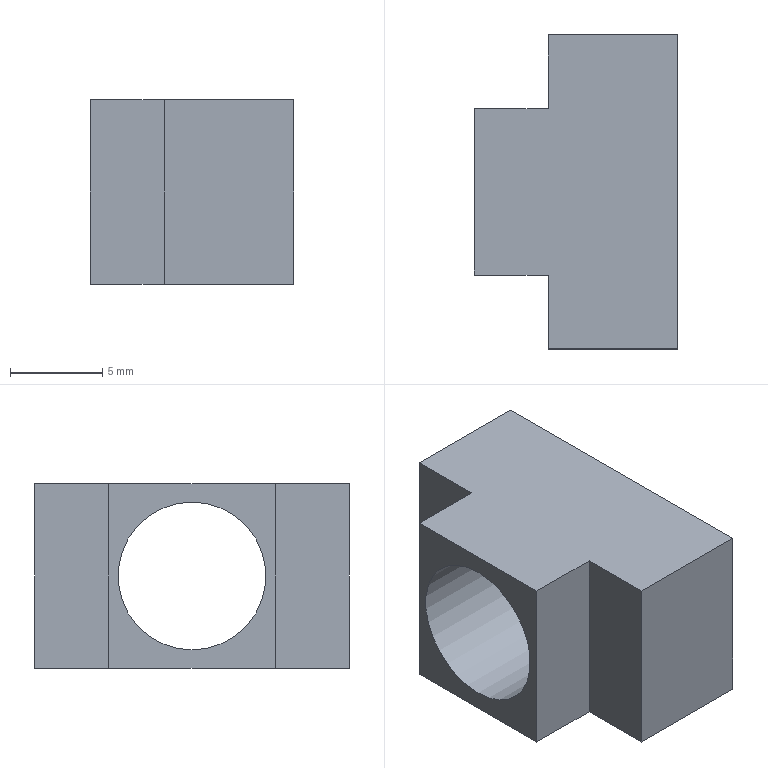Component | NX | STOP_BLOCK | 1 solid | 11 faces | box 11 x 17 x 10 mm | volume 997 mm3 | plane 10 | cylinder 1 | commonest cylinder face diameters 8 x1
STEP:
#1=CARTESIAN_POINT('',(0.,0.,0.));
#2=DIRECTION('',(0.,0.,1.));
#3=DIRECTION('',(1.,0.,0.));
#4=AXIS2_PLACEMENT_3D('',#1,#2,#3);
#5=CARTESIAN_POINT('',(-79.627,0.,11.));
#6=VERTEX_POINT('',#5);
#7=CARTESIAN_POINT('',(-79.627,0.,15.));
#8=DIRECTION('',(1.,0.,0.));
#9=DIRECTION('',(0.,0.,-1.));
#10=AXIS2_PLACEMENT_3D('',#7,#8,#9);
#11=CIRCLE('',#10,4.);
#12=CARTESIAN_POINT('',(-79.627,4.5,20.));
#13=DIRECTION('',(1.,0.,0.));
#14=DIRECTION('',(0.,0.,-1.));
#15=AXIS2_PLACEMENT_3D('',#12,#13,#14);
#16=PLANE('',#15);
#17=CARTESIAN_POINT('',(5.,-4.5));
#18=DIRECTION('',(1.,0.));
#19=AXIS2_PLACEMENT_2D('',#17,#18);
#20=CIRCLE('',#19,4.);
#21=(GEOMETRIC_REPRESENTATION_CONTEXT(2)PARAMETRIC_REPRESENTATION_CONTEXT()REPRESENTATION_CONTEXT('',''));
#22=DEFINITIONAL_REPRESENTATION('',(#20),#21);
#23=PCURVE('',#16,#22);
#24=CARTESIAN_POINT('',(-80.627,0.,15.));
#25=DIRECTION('',(1.,0.,0.));
#26=DIRECTION('',(0.,0.,-1.));
#27=AXIS2_PLACEMENT_3D('',#24,#25,#26);
#28=CYLINDRICAL_SURFACE('',#27,4.);
#29=CARTESIAN_POINT('',(0.,1.));
#30=DIRECTION('',(1.,0.));
#31=VECTOR('',#30,1.);
#32=LINE('',#29,#31);
#33=(GEOMETRIC_REPRESENTATION_CONTEXT(2)PARAMETRIC_REPRESENTATION_CONTEXT()REPRESENTATION_CONTEXT('',''));
#34=DEFINITIONAL_REPRESENTATION('',(#32),#33);
#35=PCURVE('',#28,#34);
#36=SURFACE_CURVE('',#11,(#23,#35),.PCURVE_S1.);
#37=EDGE_CURVE('',#6,#6,#36,.T.);
#38=ORIENTED_EDGE('',*,*,#37,.T.);
#39=EDGE_LOOP('',(#38));
#40=FACE_BOUND('',#39,.T.);
#41=CARTESIAN_POINT('',(-79.627,4.5,10.));
#42=VERTEX_POINT('',#41);
#43=CARTESIAN_POINT('',(-79.627,-4.5,10.));
#44=VERTEX_POINT('',#43);
#45=CARTESIAN_POINT('',(-79.627,4.5,10.));
#46=DIRECTION('',(0.,-1.,0.));
#47=VECTOR('',#46,1.);
#48=LINE('',#45,#47);
#49=CARTESIAN_POINT('',(10.,0.));
#50=DIRECTION('',(0.,-1.));
#51=VECTOR('',#50,1.);
#52=LINE('',#49,#51);
#53=(GEOMETRIC_REPRESENTATION_CONTEXT(2)PARAMETRIC_REPRESENTATION_CONTEXT()REPRESENTATION_CONTEXT('',''));
#54=DEFINITIONAL_REPRESENTATION('',(#52),#53);
#55=PCURVE('',#16,#54);
#56=CARTESIAN_POINT('',(-79.627,0.,10.));
#57=DIRECTION('',(0.,0.,1.));
#58=DIRECTION('',(1.,0.,0.));
#59=AXIS2_PLACEMENT_3D('',#56,#57,#58);
#60=PLANE('',#59);
#61=CARTESIAN_POINT('',(0.,4.5));
#62=DIRECTION('',(0.,-1.));
#63=VECTOR('',#62,1.);
#64=LINE('',#61,#63);
#65=(GEOMETRIC_REPRESENTATION_CONTEXT(2)PARAMETRIC_REPRESENTATION_CONTEXT()REPRESENTATION_CONTEXT('',''));
#66=DEFINITIONAL_REPRESENTATION('',(#64),#65);
#67=PCURVE('',#60,#66);
#68=SURFACE_CURVE('',#48,(#55,#67),.PCURVE_S1.);
#69=EDGE_CURVE('',#42,#44,#68,.T.);
#70=ORIENTED_EDGE('',*,*,#69,.T.);
#71=CARTESIAN_POINT('',(-79.627,-4.5,20.));
#72=VERTEX_POINT('',#71);
#73=CARTESIAN_POINT('',(-79.627,-4.5,20.));
#74=DIRECTION('',(0.,0.,-1.));
#75=VECTOR('',#74,1.);
#76=LINE('',#73,#75);
#77=CARTESIAN_POINT('',(0.,-9.));
#78=DIRECTION('',(1.,0.));
#79=VECTOR('',#78,1.);
#80=LINE('',#77,#79);
#81=(GEOMETRIC_REPRESENTATION_CONTEXT(2)PARAMETRIC_REPRESENTATION_CONTEXT()REPRESENTATION_CONTEXT('',''));
#82=DEFINITIONAL_REPRESENTATION('',(#80),#81);
#83=PCURVE('',#16,#82);
#84=CARTESIAN_POINT('',(-79.627,-4.5,20.));
#85=DIRECTION('',(0.,1.,0.));
#86=DIRECTION('',(0.,0.,1.));
#87=AXIS2_PLACEMENT_3D('',#84,#85,#86);
#88=PLANE('',#87);
#89=CARTESIAN_POINT('',(0.,0.));
#90=DIRECTION('',(-1.,0.));
#91=VECTOR('',#90,1.);
#92=LINE('',#89,#91);
#93=(GEOMETRIC_REPRESENTATION_CONTEXT(2)PARAMETRIC_REPRESENTATION_CONTEXT()REPRESENTATION_CONTEXT('',''));
#94=DEFINITIONAL_REPRESENTATION('',(#92),#93);
#95=PCURVE('',#88,#94);
#96=SURFACE_CURVE('',#76,(#83,#95),.PCURVE_S1.);
#97=EDGE_CURVE('',#72,#44,#96,.T.);
#98=ORIENTED_EDGE('',*,*,#97,.F.);
#99=CARTESIAN_POINT('',(-79.627,4.5,20.));
#100=VERTEX_POINT('',#99);
#101=CARTESIAN_POINT('',(-79.627,4.5,20.));
#102=DIRECTION('',(0.,-1.,0.));
#103=VECTOR('',#102,1.);
#104=LINE('',#101,#103);
#105=CARTESIAN_POINT('',(0.,0.));
#106=DIRECTION('',(0.,-1.));
#107=VECTOR('',#106,1.);
#108=LINE('',#105,#107);
#109=(GEOMETRIC_REPRESENTATION_CONTEXT(2)PARAMETRIC_REPRESENTATION_CONTEXT()REPRESENTATION_CONTEXT('',''));
#110=DEFINITIONAL_REPRESENTATION('',(#108),#109);
#111=PCURVE('',#16,#110);
#112=CARTESIAN_POINT('',(-79.627,0.,20.));
#113=DIRECTION('',(0.,0.,1.));
#114=DIRECTION('',(1.,0.,0.));
#115=AXIS2_PLACEMENT_3D('',#112,#113,#114);
#116=PLANE('',#115);
#117=CARTESIAN_POINT('',(0.,4.5));
#118=DIRECTION('',(0.,-1.));
#119=VECTOR('',#118,1.);
#120=LINE('',#117,#119);
#121=(GEOMETRIC_REPRESENTATION_CONTEXT(2)PARAMETRIC_REPRESENTATION_CONTEXT()REPRESENTATION_CONTEXT('',''));
#122=DEFINITIONAL_REPRESENTATION('',(#120),#121);
#123=PCURVE('',#116,#122);
#124=SURFACE_CURVE('',#104,(#111,#123),.PCURVE_S1.);
#125=EDGE_CURVE('',#100,#72,#124,.T.);
#126=ORIENTED_EDGE('',*,*,#125,.F.);
#127=CARTESIAN_POINT('',(-79.627,4.5,20.));
#128=DIRECTION('',(0.,0.,-1.));
#129=VECTOR('',#128,1.);
#130=LINE('',#127,#129);
#131=CARTESIAN_POINT('',(0.,0.));
#132=DIRECTION('',(1.,0.));
#133=VECTOR('',#132,1.);
#134=LINE('',#131,#133);
#135=(GEOMETRIC_REPRESENTATION_CONTEXT(2)PARAMETRIC_REPRESENTATION_CONTEXT()REPRESENTATION_CONTEXT('',''));
#136=DEFINITIONAL_REPRESENTATION('',(#134),#135);
#137=PCURVE('',#16,#136);
#138=CARTESIAN_POINT('',(-75.627,4.5,20.));
#139=DIRECTION('',(0.,-1.,0.));
#140=DIRECTION('',(0.,0.,-1.));
#141=AXIS2_PLACEMENT_3D('',#138,#139,#140);
#142=PLANE('',#141);
#143=CARTESIAN_POINT('',(0.,-4.));
#144=DIRECTION('',(1.,0.));
#145=VECTOR('',#144,1.);
#146=LINE('',#143,#145);
#147=(GEOMETRIC_REPRESENTATION_CONTEXT(2)PARAMETRIC_REPRESENTATION_CONTEXT()REPRESENTATION_CONTEXT('',''));
#148=DEFINITIONAL_REPRESENTATION('',(#146),#147);
#149=PCURVE('',#142,#148);
#150=SURFACE_CURVE('',#130,(#137,#149),.PCURVE_S1.);
#151=EDGE_CURVE('',#100,#42,#150,.T.);
#152=ORIENTED_EDGE('',*,*,#151,.T.);
#153=EDGE_LOOP('',(#70,#98,#126,#152));
#154=FACE_BOUND('',#153,.T.);
#155=ADVANCED_FACE('',(#40,#154),#16,.F.);
#156=CARTESIAN_POINT('',(-75.627,-4.5,10.));
#157=VERTEX_POINT('',#156);
#158=CARTESIAN_POINT('',(-79.627,-4.5,10.));
#159=DIRECTION('',(1.,0.,0.));
#160=VECTOR('',#159,1.);
#161=LINE('',#158,#160);
#162=CARTESIAN_POINT('',(-10.,0.));
#163=DIRECTION('',(0.,1.));
#164=VECTOR('',#163,1.);
#165=LINE('',#162,#164);
#166=(GEOMETRIC_REPRESENTATION_CONTEXT(2)PARAMETRIC_REPRESENTATION_CONTEXT()REPRESENTATION_CONTEXT('',''));
#167=DEFINITIONAL_REPRESENTATION('',(#165),#166);
#168=PCURVE('',#88,#167);
#169=CARTESIAN_POINT('',(0.,-4.5));
#170=DIRECTION('',(1.,0.));
#171=VECTOR('',#170,1.);
#172=LINE('',#169,#171);
#173=(GEOMETRIC_REPRESENTATION_CONTEXT(2)PARAMETRIC_REPRESENTATION_CONTEXT()REPRESENTATION_CONTEXT('',''));
#174=DEFINITIONAL_REPRESENTATION('',(#172),#173);
#175=PCURVE('',#60,#174);
#176=SURFACE_CURVE('',#161,(#168,#175),.PCURVE_S1.);
#177=EDGE_CURVE('',#44,#157,#176,.T.);
#178=ORIENTED_EDGE('',*,*,#177,.T.);
#179=CARTESIAN_POINT('',(-75.627,-4.5,20.));
#180=VERTEX_POINT('',#179);
#181=CARTESIAN_POINT('',(-75.627,-4.5,20.));
#182=DIRECTION('',(0.,0.,-1.));
#183=VECTOR('',#182,1.);
#184=LINE('',#181,#183);
#185=CARTESIAN_POINT('',(0.,4.));
#186=DIRECTION('',(-1.,0.));
#187=VECTOR('',#186,1.);
#188=LINE('',#185,#187);
#189=(GEOMETRIC_REPRESENTATION_CONTEXT(2)PARAMETRIC_REPRESENTATION_CONTEXT()REPRESENTATION_CONTEXT('',''));
#190=DEFINITIONAL_REPRESENTATION('',(#188),#189);
#191=PCURVE('',#88,#190);
#192=CARTESIAN_POINT('',(-75.627,-4.5,20.));
#193=DIRECTION('',(1.,0.,0.));
#194=DIRECTION('',(0.,0.,-1.));
#195=AXIS2_PLACEMENT_3D('',#192,#193,#194);
#196=PLANE('',#195);
#197=CARTESIAN_POINT('',(0.,0.));
#198=DIRECTION('',(1.,0.));
#199=VECTOR('',#198,1.);
#200=LINE('',#197,#199);
#201=(GEOMETRIC_REPRESENTATION_CONTEXT(2)PARAMETRIC_REPRESENTATION_CONTEXT()REPRESENTATION_CONTEXT('',''));
#202=DEFINITIONAL_REPRESENTATION('',(#200),#201);
#203=PCURVE('',#196,#202);
#204=SURFACE_CURVE('',#184,(#191,#203),.PCURVE_S1.);
#205=EDGE_CURVE('',#180,#157,#204,.T.);
#206=ORIENTED_EDGE('',*,*,#205,.F.);
#207=CARTESIAN_POINT('',(-79.627,-4.5,20.));
#208=DIRECTION('',(1.,0.,0.));
#209=VECTOR('',#208,1.);
#210=LINE('',#207,#209);
#211=CARTESIAN_POINT('',(0.,0.));
#212=DIRECTION('',(0.,1.));
#213=VECTOR('',#212,1.);
#214=LINE('',#211,#213);
#215=(GEOMETRIC_REPRESENTATION_CONTEXT(2)PARAMETRIC_REPRESENTATION_CONTEXT()REPRESENTATION_CONTEXT('',''));
#216=DEFINITIONAL_REPRESENTATION('',(#214),#215);
#217=PCURVE('',#88,#216);
#218=CARTESIAN_POINT('',(0.,-4.5));
#219=DIRECTION('',(1.,0.));
#220=VECTOR('',#219,1.);
#221=LINE('',#218,#220);
#222=(GEOMETRIC_REPRESENTATION_CONTEXT(2)PARAMETRIC_REPRESENTATION_CONTEXT()REPRESENTATION_CONTEXT('',''));
#223=DEFINITIONAL_REPRESENTATION('',(#221),#222);
#224=PCURVE('',#116,#223);
#225=SURFACE_CURVE('',#210,(#217,#224),.PCURVE_S1.);
#226=EDGE_CURVE('',#72,#180,#225,.T.);
#227=ORIENTED_EDGE('',*,*,#226,.F.);
#228=ORIENTED_EDGE('',*,*,#97,.T.);
#229=EDGE_LOOP('',(#178,#206,#227,#228));
#230=FACE_BOUND('',#229,.T.);
#231=ADVANCED_FACE('',(#230),#88,.F.);
#232=CARTESIAN_POINT('',(-75.627,-8.5,10.));
#233=VERTEX_POINT('',#232);
#234=CARTESIAN_POINT('',(-75.627,-4.5,10.));
#235=DIRECTION('',(0.,-1.,0.));
#236=VECTOR('',#235,1.);
#237=LINE('',#234,#236);
#238=CARTESIAN_POINT('',(10.,0.));
#239=DIRECTION('',(0.,-1.));
#240=VECTOR('',#239,1.);
#241=LINE('',#238,#240);
#242=(GEOMETRIC_REPRESENTATION_CONTEXT(2)PARAMETRIC_REPRESENTATION_CONTEXT()REPRESENTATION_CONTEXT('',''));
#243=DEFINITIONAL_REPRESENTATION('',(#241),#242);
#244=PCURVE('',#196,#243);
#245=CARTESIAN_POINT('',(4.,-4.5));
#246=DIRECTION('',(0.,-1.));
#247=VECTOR('',#246,1.);
#248=LINE('',#245,#247);
#249=(GEOMETRIC_REPRESENTATION_CONTEXT(2)PARAMETRIC_REPRESENTATION_CONTEXT()REPRESENTATION_CONTEXT('',''));
#250=DEFINITIONAL_REPRESENTATION('',(#248),#249);
#251=PCURVE('',#60,#250);
#252=SURFACE_CURVE('',#237,(#244,#251),.PCURVE_S1.);
#253=EDGE_CURVE('',#157,#233,#252,.T.);
#254=ORIENTED_EDGE('',*,*,#253,.T.);
#255=CARTESIAN_POINT('',(-75.627,-8.5,20.));
#256=VERTEX_POINT('',#255);
#257=CARTESIAN_POINT('',(-75.627,-8.5,20.));
#258=DIRECTION('',(0.,0.,-1.));
#259=VECTOR('',#258,1.);
#260=LINE('',#257,#259);
#261=CARTESIAN_POINT('',(0.,-4.));
#262=DIRECTION('',(1.,0.));
#263=VECTOR('',#262,1.);
#264=LINE('',#261,#263);
#265=(GEOMETRIC_REPRESENTATION_CONTEXT(2)PARAMETRIC_REPRESENTATION_CONTEXT()REPRESENTATION_CONTEXT('',''));
#266=DEFINITIONAL_REPRESENTATION('',(#264),#265);
#267=PCURVE('',#196,#266);
#268=CARTESIAN_POINT('',(-75.627,-8.5,20.));
#269=DIRECTION('',(0.,1.,0.));
#270=DIRECTION('',(0.,0.,1.));
#271=AXIS2_PLACEMENT_3D('',#268,#269,#270);
#272=PLANE('',#271);
#273=CARTESIAN_POINT('',(0.,0.));
#274=DIRECTION('',(-1.,0.));
#275=VECTOR('',#274,1.);
#276=LINE('',#273,#275);
#277=(GEOMETRIC_REPRESENTATION_CONTEXT(2)PARAMETRIC_REPRESENTATION_CONTEXT()REPRESENTATION_CONTEXT('',''));
#278=DEFINITIONAL_REPRESENTATION('',(#276),#277);
#279=PCURVE('',#272,#278);
#280=SURFACE_CURVE('',#260,(#267,#279),.PCURVE_S1.);
#281=EDGE_CURVE('',#256,#233,#280,.T.);
#282=ORIENTED_EDGE('',*,*,#281,.F.);
#283=CARTESIAN_POINT('',(-75.627,-4.5,20.));
#284=DIRECTION('',(0.,-1.,0.));
#285=VECTOR('',#284,1.);
#286=LINE('',#283,#285);
#287=CARTESIAN_POINT('',(0.,0.));
#288=DIRECTION('',(0.,-1.));
#289=VECTOR('',#288,1.);
#290=LINE('',#287,#289);
#291=(GEOMETRIC_REPRESENTATION_CONTEXT(2)PARAMETRIC_REPRESENTATION_CONTEXT()REPRESENTATION_CONTEXT('',''));
#292=DEFINITIONAL_REPRESENTATION('',(#290),#291);
#293=PCURVE('',#196,#292);
#294=CARTESIAN_POINT('',(4.,-4.5));
#295=DIRECTION('',(0.,-1.));
#296=VECTOR('',#295,1.);
#297=LINE('',#294,#296);
#298=(GEOMETRIC_REPRESENTATION_CONTEXT(2)PARAMETRIC_REPRESENTATION_CONTEXT()REPRESENTATION_CONTEXT('',''));
#299=DEFINITIONAL_REPRESENTATION('',(#297),#298);
#300=PCURVE('',#116,#299);
#301=SURFACE_CURVE('',#286,(#293,#300),.PCURVE_S1.);
#302=EDGE_CURVE('',#180,#256,#301,.T.);
#303=ORIENTED_EDGE('',*,*,#302,.F.);
#304=ORIENTED_EDGE('',*,*,#205,.T.);
#305=EDGE_LOOP('',(#254,#282,#303,#304));
#306=FACE_BOUND('',#305,.T.);
#307=ADVANCED_FACE('',(#306),#196,.F.);
#308=CARTESIAN_POINT('',(-68.627,-8.5,10.));
#309=VERTEX_POINT('',#308);
#310=CARTESIAN_POINT('',(-75.627,-8.5,10.));
#311=DIRECTION('',(1.,0.,0.));
#312=VECTOR('',#311,1.);
#313=LINE('',#310,#312);
#314=CARTESIAN_POINT('',(-10.,0.));
#315=DIRECTION('',(0.,1.));
#316=VECTOR('',#315,1.);
#317=LINE('',#314,#316);
#318=(GEOMETRIC_REPRESENTATION_CONTEXT(2)PARAMETRIC_REPRESENTATION_CONTEXT()REPRESENTATION_CONTEXT('',''));
#319=DEFINITIONAL_REPRESENTATION('',(#317),#318);
#320=PCURVE('',#272,#319);
#321=CARTESIAN_POINT('',(4.,-8.5));
#322=DIRECTION('',(1.,0.));
#323=VECTOR('',#322,1.);
#324=LINE('',#321,#323);
#325=(GEOMETRIC_REPRESENTATION_CONTEXT(2)PARAMETRIC_REPRESENTATION_CONTEXT()REPRESENTATION_CONTEXT('',''));
#326=DEFINITIONAL_REPRESENTATION('',(#324),#325);
#327=PCURVE('',#60,#326);
#328=SURFACE_CURVE('',#313,(#320,#327),.PCURVE_S1.);
#329=EDGE_CURVE('',#233,#309,#328,.T.);
#330=ORIENTED_EDGE('',*,*,#329,.T.);
#331=CARTESIAN_POINT('',(-68.627,-8.5,20.));
#332=VERTEX_POINT('',#331);
#333=CARTESIAN_POINT('',(-68.627,-8.5,20.));
#334=DIRECTION('',(0.,0.,-1.));
#335=VECTOR('',#334,1.);
#336=LINE('',#333,#335);
#337=CARTESIAN_POINT('',(0.,7.));
#338=DIRECTION('',(-1.,0.));
#339=VECTOR('',#338,1.);
#340=LINE('',#337,#339);
#341=(GEOMETRIC_REPRESENTATION_CONTEXT(2)PARAMETRIC_REPRESENTATION_CONTEXT()REPRESENTATION_CONTEXT('',''));
#342=DEFINITIONAL_REPRESENTATION('',(#340),#341);
#343=PCURVE('',#272,#342);
#344=CARTESIAN_POINT('',(-68.627,-8.5,20.));
#345=DIRECTION('',(-1.,0.,0.));
#346=DIRECTION('',(0.,0.,1.));
#347=AXIS2_PLACEMENT_3D('',#344,#345,#346);
#348=PLANE('',#347);
#349=CARTESIAN_POINT('',(0.,0.));
#350=DIRECTION('',(-1.,0.));
#351=VECTOR('',#350,1.);
#352=LINE('',#349,#351);
#353=(GEOMETRIC_REPRESENTATION_CONTEXT(2)PARAMETRIC_REPRESENTATION_CONTEXT()REPRESENTATION_CONTEXT('',''));
#354=DEFINITIONAL_REPRESENTATION('',(#352),#353);
#355=PCURVE('',#348,#354);
#356=SURFACE_CURVE('',#336,(#343,#355),.PCURVE_S1.);
#357=EDGE_CURVE('',#332,#309,#356,.T.);
#358=ORIENTED_EDGE('',*,*,#357,.F.);
#359=CARTESIAN_POINT('',(-75.627,-8.5,20.));
#360=DIRECTION('',(1.,0.,0.));
#361=VECTOR('',#360,1.);
#362=LINE('',#359,#361);
#363=CARTESIAN_POINT('',(0.,0.));
#364=DIRECTION('',(0.,1.));
#365=VECTOR('',#364,1.);
#366=LINE('',#363,#365);
#367=(GEOMETRIC_REPRESENTATION_CONTEXT(2)PARAMETRIC_REPRESENTATION_CONTEXT()REPRESENTATION_CONTEXT('',''));
#368=DEFINITIONAL_REPRESENTATION('',(#366),#367);
#369=PCURVE('',#272,#368);
#370=CARTESIAN_POINT('',(4.,-8.5));
#371=DIRECTION('',(1.,0.));
#372=VECTOR('',#371,1.);
#373=LINE('',#370,#372);
#374=(GEOMETRIC_REPRESENTATION_CONTEXT(2)PARAMETRIC_REPRESENTATION_CONTEXT()REPRESENTATION_CONTEXT('',''));
#375=DEFINITIONAL_REPRESENTATION('',(#373),#374);
#376=PCURVE('',#116,#375);
#377=SURFACE_CURVE('',#362,(#369,#376),.PCURVE_S1.);
#378=EDGE_CURVE('',#256,#332,#377,.T.);
#379=ORIENTED_EDGE('',*,*,#378,.F.);
#380=ORIENTED_EDGE('',*,*,#281,.T.);
#381=EDGE_LOOP('',(#330,#358,#379,#380));
#382=FACE_BOUND('',#381,.T.);
#383=ADVANCED_FACE('',(#382),#272,.F.);
#384=CARTESIAN_POINT('',(-68.627,0.,19.));
#385=VERTEX_POINT('',#384);
#386=CARTESIAN_POINT('',(-68.627,0.,11.));
#387=VERTEX_POINT('',#386);
#388=CARTESIAN_POINT('',(-68.627,0.,15.));
#389=DIRECTION('',(-1.,0.,0.));
#390=DIRECTION('',(0.,0.,1.));
#391=AXIS2_PLACEMENT_3D('',#388,#389,#390);
#392=CIRCLE('',#391,4.);
#393=CARTESIAN_POINT('',(-5.,8.5));
#394=DIRECTION('',(1.,0.));
#395=AXIS2_PLACEMENT_2D('',#393,#394);
#396=CIRCLE('',#395,4.);
#397=(GEOMETRIC_REPRESENTATION_CONTEXT(2)PARAMETRIC_REPRESENTATION_CONTEXT()REPRESENTATION_CONTEXT('',''));
#398=DEFINITIONAL_REPRESENTATION('',(#396),#397);
#399=PCURVE('',#348,#398);
#400=CARTESIAN_POINT('',(3.142,12.));
#401=DIRECTION('',(-1.,0.));
#402=VECTOR('',#401,1.);
#403=LINE('',#400,#402);
#404=(GEOMETRIC_REPRESENTATION_CONTEXT(2)PARAMETRIC_REPRESENTATION_CONTEXT()REPRESENTATION_CONTEXT('',''));
#405=DEFINITIONAL_REPRESENTATION('',(#403),#404);
#406=PCURVE('',#28,#405);
#407=SURFACE_CURVE('',#392,(#399,#406),.PCURVE_S1.);
#408=EDGE_CURVE('',#385,#387,#407,.T.);
#409=ORIENTED_EDGE('',*,*,#408,.T.);
#410=CARTESIAN_POINT('',(-68.627,0.,15.));
#411=DIRECTION('',(-1.,0.,0.));
#412=DIRECTION('',(0.,0.,1.));
#413=AXIS2_PLACEMENT_3D('',#410,#411,#412);
#414=CIRCLE('',#413,4.);
#415=CARTESIAN_POINT('',(-5.,8.5));
#416=DIRECTION('',(1.,0.));
#417=AXIS2_PLACEMENT_2D('',#415,#416);
#418=CIRCLE('',#417,4.);
#419=(GEOMETRIC_REPRESENTATION_CONTEXT(2)PARAMETRIC_REPRESENTATION_CONTEXT()REPRESENTATION_CONTEXT('',''));
#420=DEFINITIONAL_REPRESENTATION('',(#418),#419);
#421=PCURVE('',#348,#420);
#422=CARTESIAN_POINT('',(9.425,12.));
#423=DIRECTION('',(-1.,0.));
#424=VECTOR('',#423,1.);
#425=LINE('',#422,#424);
#426=(GEOMETRIC_REPRESENTATION_CONTEXT(2)PARAMETRIC_REPRESENTATION_CONTEXT()REPRESENTATION_CONTEXT('',''));
#427=DEFINITIONAL_REPRESENTATION('',(#425),#426);
#428=PCURVE('',#28,#427);
#429=SURFACE_CURVE('',#414,(#421,#428),.PCURVE_S1.);
#430=EDGE_CURVE('',#387,#385,#429,.T.);
#431=ORIENTED_EDGE('',*,*,#430,.T.);
#432=EDGE_LOOP('',(#409,#431));
#433=FACE_BOUND('',#432,.T.);
#434=CARTESIAN_POINT('',(-68.627,8.5,10.));
#435=VERTEX_POINT('',#434);
#436=CARTESIAN_POINT('',(-68.627,-8.5,10.));
#437=DIRECTION('',(0.,1.,0.));
#438=VECTOR('',#437,1.);
#439=LINE('',#436,#438);
#440=CARTESIAN_POINT('',(-10.,0.));
#441=DIRECTION('',(0.,1.));
#442=VECTOR('',#441,1.);
#443=LINE('',#440,#442);
#444=(GEOMETRIC_REPRESENTATION_CONTEXT(2)PARAMETRIC_REPRESENTATION_CONTEXT()REPRESENTATION_CONTEXT('',''));
#445=DEFINITIONAL_REPRESENTATION('',(#443),#444);
#446=PCURVE('',#348,#445);
#447=CARTESIAN_POINT('',(11.,-8.5));
#448=DIRECTION('',(0.,1.));
#449=VECTOR('',#448,1.);
#450=LINE('',#447,#449);
#451=(GEOMETRIC_REPRESENTATION_CONTEXT(2)PARAMETRIC_REPRESENTATION_CONTEXT()REPRESENTATION_CONTEXT('',''));
#452=DEFINITIONAL_REPRESENTATION('',(#450),#451);
#453=PCURVE('',#60,#452);
#454=SURFACE_CURVE('',#439,(#446,#453),.PCURVE_S1.);
#455=EDGE_CURVE('',#309,#435,#454,.T.);
#456=ORIENTED_EDGE('',*,*,#455,.T.);
#457=CARTESIAN_POINT('',(-68.627,8.5,20.));
#458=VERTEX_POINT('',#457);
#459=CARTESIAN_POINT('',(-68.627,8.5,20.));
#460=DIRECTION('',(0.,0.,-1.));
#461=VECTOR('',#460,1.);
#462=LINE('',#459,#461);
#463=CARTESIAN_POINT('',(0.,17.));
#464=DIRECTION('',(-1.,0.));
#465=VECTOR('',#464,1.);
#466=LINE('',#463,#465);
#467=(GEOMETRIC_REPRESENTATION_CONTEXT(2)PARAMETRIC_REPRESENTATION_CONTEXT()REPRESENTATION_CONTEXT('',''));
#468=DEFINITIONAL_REPRESENTATION('',(#466),#467);
#469=PCURVE('',#348,#468);
#470=CARTESIAN_POINT('',(-68.627,8.5,20.));
#471=DIRECTION('',(0.,-1.,0.));
#472=DIRECTION('',(0.,0.,-1.));
#473=AXIS2_PLACEMENT_3D('',#470,#471,#472);
#474=PLANE('',#473);
#475=CARTESIAN_POINT('',(0.,0.));
#476=DIRECTION('',(1.,0.));
#477=VECTOR('',#476,1.);
#478=LINE('',#475,#477);
#479=(GEOMETRIC_REPRESENTATION_CONTEXT(2)PARAMETRIC_REPRESENTATION_CONTEXT()REPRESENTATION_CONTEXT('',''));
#480=DEFINITIONAL_REPRESENTATION('',(#478),#479);
#481=PCURVE('',#474,#480);
#482=SURFACE_CURVE('',#462,(#469,#481),.PCURVE_S1.);
#483=EDGE_CURVE('',#458,#435,#482,.T.);
#484=ORIENTED_EDGE('',*,*,#483,.F.);
#485=CARTESIAN_POINT('',(-68.627,-8.5,20.));
#486=DIRECTION('',(0.,1.,0.));
#487=VECTOR('',#486,1.);
#488=LINE('',#485,#487);
#489=CARTESIAN_POINT('',(0.,0.));
#490=DIRECTION('',(0.,1.));
#491=VECTOR('',#490,1.);
#492=LINE('',#489,#491);
#493=(GEOMETRIC_REPRESENTATION_CONTEXT(2)PARAMETRIC_REPRESENTATION_CONTEXT()REPRESENTATION_CONTEXT('',''));
#494=DEFINITIONAL_REPRESENTATION('',(#492),#493);
#495=PCURVE('',#348,#494);
#496=CARTESIAN_POINT('',(11.,-8.5));
#497=DIRECTION('',(0.,1.));
#498=VECTOR('',#497,1.);
#499=LINE('',#496,#498);
#500=(GEOMETRIC_REPRESENTATION_CONTEXT(2)PARAMETRIC_REPRESENTATION_CONTEXT()REPRESENTATION_CONTEXT('',''));
#501=DEFINITIONAL_REPRESENTATION('',(#499),#500);
#502=PCURVE('',#116,#501);
#503=SURFACE_CURVE('',#488,(#495,#502),.PCURVE_S1.);
#504=EDGE_CURVE('',#332,#458,#503,.T.);
#505=ORIENTED_EDGE('',*,*,#504,.F.);
#506=ORIENTED_EDGE('',*,*,#357,.T.);
#507=EDGE_LOOP('',(#456,#484,#505,#506));
#508=FACE_BOUND('',#507,.T.);
#509=ADVANCED_FACE('',(#433,#508),#348,.F.);
#510=CARTESIAN_POINT('',(-75.627,8.5,10.));
#511=VERTEX_POINT('',#510);
#512=CARTESIAN_POINT('',(-68.627,8.5,10.));
#513=DIRECTION('',(-1.,0.,0.));
#514=VECTOR('',#513,1.);
#515=LINE('',#512,#514);
#516=CARTESIAN_POINT('',(10.,0.));
#517=DIRECTION('',(0.,-1.));
#518=VECTOR('',#517,1.);
#519=LINE('',#516,#518);
#520=(GEOMETRIC_REPRESENTATION_CONTEXT(2)PARAMETRIC_REPRESENTATION_CONTEXT()REPRESENTATION_CONTEXT('',''));
#521=DEFINITIONAL_REPRESENTATION('',(#519),#520);
#522=PCURVE('',#474,#521);
#523=CARTESIAN_POINT('',(11.,8.5));
#524=DIRECTION('',(-1.,0.));
#525=VECTOR('',#524,1.);
#526=LINE('',#523,#525);
#527=(GEOMETRIC_REPRESENTATION_CONTEXT(2)PARAMETRIC_REPRESENTATION_CONTEXT()REPRESENTATION_CONTEXT('',''));
#528=DEFINITIONAL_REPRESENTATION('',(#526),#527);
#529=PCURVE('',#60,#528);
#530=SURFACE_CURVE('',#515,(#522,#529),.PCURVE_S1.);
#531=EDGE_CURVE('',#435,#511,#530,.T.);
#532=ORIENTED_EDGE('',*,*,#531,.T.);
#533=CARTESIAN_POINT('',(-75.627,8.5,20.));
#534=VERTEX_POINT('',#533);
#535=CARTESIAN_POINT('',(-75.627,8.5,20.));
#536=DIRECTION('',(0.,0.,-1.));
#537=VECTOR('',#536,1.);
#538=LINE('',#535,#537);
#539=CARTESIAN_POINT('',(0.,-7.));
#540=DIRECTION('',(1.,0.));
#541=VECTOR('',#540,1.);
#542=LINE('',#539,#541);
#543=(GEOMETRIC_REPRESENTATION_CONTEXT(2)PARAMETRIC_REPRESENTATION_CONTEXT()REPRESENTATION_CONTEXT('',''));
#544=DEFINITIONAL_REPRESENTATION('',(#542),#543);
#545=PCURVE('',#474,#544);
#546=CARTESIAN_POINT('',(-75.627,8.5,20.));
#547=DIRECTION('',(1.,0.,0.));
#548=DIRECTION('',(0.,0.,-1.));
#549=AXIS2_PLACEMENT_3D('',#546,#547,#548);
#550=PLANE('',#549);
#551=CARTESIAN_POINT('',(0.,0.));
#552=DIRECTION('',(1.,0.));
#553=VECTOR('',#552,1.);
#554=LINE('',#551,#553);
#555=(GEOMETRIC_REPRESENTATION_CONTEXT(2)PARAMETRIC_REPRESENTATION_CONTEXT()REPRESENTATION_CONTEXT('',''));
#556=DEFINITIONAL_REPRESENTATION('',(#554),#555);
#557=PCURVE('',#550,#556);
#558=SURFACE_CURVE('',#538,(#545,#557),.PCURVE_S1.);
#559=EDGE_CURVE('',#534,#511,#558,.T.);
#560=ORIENTED_EDGE('',*,*,#559,.F.);
#561=CARTESIAN_POINT('',(-68.627,8.5,20.));
#562=DIRECTION('',(-1.,0.,0.));
#563=VECTOR('',#562,1.);
#564=LINE('',#561,#563);
#565=CARTESIAN_POINT('',(0.,0.));
#566=DIRECTION('',(0.,-1.));
#567=VECTOR('',#566,1.);
#568=LINE('',#565,#567);
#569=(GEOMETRIC_REPRESENTATION_CONTEXT(2)PARAMETRIC_REPRESENTATION_CONTEXT()REPRESENTATION_CONTEXT('',''));
#570=DEFINITIONAL_REPRESENTATION('',(#568),#569);
#571=PCURVE('',#474,#570);
#572=CARTESIAN_POINT('',(11.,8.5));
#573=DIRECTION('',(-1.,0.));
#574=VECTOR('',#573,1.);
#575=LINE('',#572,#574);
#576=(GEOMETRIC_REPRESENTATION_CONTEXT(2)PARAMETRIC_REPRESENTATION_CONTEXT()REPRESENTATION_CONTEXT('',''));
#577=DEFINITIONAL_REPRESENTATION('',(#575),#576);
#578=PCURVE('',#116,#577);
#579=SURFACE_CURVE('',#564,(#571,#578),.PCURVE_S1.);
#580=EDGE_CURVE('',#458,#534,#579,.T.);
#581=ORIENTED_EDGE('',*,*,#580,.F.);
#582=ORIENTED_EDGE('',*,*,#483,.T.);
#583=EDGE_LOOP('',(#532,#560,#581,#582));
#584=FACE_BOUND('',#583,.T.);
#585=ADVANCED_FACE('',(#584),#474,.F.);
#586=CARTESIAN_POINT('',(-75.627,4.5,10.));
#587=VERTEX_POINT('',#586);
#588=CARTESIAN_POINT('',(-75.627,8.5,10.));
#589=DIRECTION('',(0.,-1.,0.));
#590=VECTOR('',#589,1.);
#591=LINE('',#588,#590);
#592=CARTESIAN_POINT('',(10.,0.));
#593=DIRECTION('',(0.,-1.));
#594=VECTOR('',#593,1.);
#595=LINE('',#592,#594);
#596=(GEOMETRIC_REPRESENTATION_CONTEXT(2)PARAMETRIC_REPRESENTATION_CONTEXT()REPRESENTATION_CONTEXT('',''));
#597=DEFINITIONAL_REPRESENTATION('',(#595),#596);
#598=PCURVE('',#550,#597);
#599=CARTESIAN_POINT('',(4.,8.5));
#600=DIRECTION('',(0.,-1.));
#601=VECTOR('',#600,1.);
#602=LINE('',#599,#601);
#603=(GEOMETRIC_REPRESENTATION_CONTEXT(2)PARAMETRIC_REPRESENTATION_CONTEXT()REPRESENTATION_CONTEXT('',''));
#604=DEFINITIONAL_REPRESENTATION('',(#602),#603);
#605=PCURVE('',#60,#604);
#606=SURFACE_CURVE('',#591,(#598,#605),.PCURVE_S1.);
#607=EDGE_CURVE('',#511,#587,#606,.T.);
#608=ORIENTED_EDGE('',*,*,#607,.T.);
#609=CARTESIAN_POINT('',(-75.627,4.5,20.));
#610=VERTEX_POINT('',#609);
#611=CARTESIAN_POINT('',(-75.627,4.5,20.));
#612=DIRECTION('',(0.,0.,-1.));
#613=VECTOR('',#612,1.);
#614=LINE('',#611,#613);
#615=CARTESIAN_POINT('',(0.,-4.));
#616=DIRECTION('',(1.,0.));
#617=VECTOR('',#616,1.);
#618=LINE('',#615,#617);
#619=(GEOMETRIC_REPRESENTATION_CONTEXT(2)PARAMETRIC_REPRESENTATION_CONTEXT()REPRESENTATION_CONTEXT('',''));
#620=DEFINITIONAL_REPRESENTATION('',(#618),#619);
#621=PCURVE('',#550,#620);
#622=CARTESIAN_POINT('',(0.,0.));
#623=DIRECTION('',(1.,0.));
#624=VECTOR('',#623,1.);
#625=LINE('',#622,#624);
#626=(GEOMETRIC_REPRESENTATION_CONTEXT(2)PARAMETRIC_REPRESENTATION_CONTEXT()REPRESENTATION_CONTEXT('',''));
#627=DEFINITIONAL_REPRESENTATION('',(#625),#626);
#628=PCURVE('',#142,#627);
#629=SURFACE_CURVE('',#614,(#621,#628),.PCURVE_S1.);
#630=EDGE_CURVE('',#610,#587,#629,.T.);
#631=ORIENTED_EDGE('',*,*,#630,.F.);
#632=CARTESIAN_POINT('',(-75.627,8.5,20.));
#633=DIRECTION('',(0.,-1.,0.));
#634=VECTOR('',#633,1.);
#635=LINE('',#632,#634);
#636=CARTESIAN_POINT('',(0.,0.));
#637=DIRECTION('',(0.,-1.));
#638=VECTOR('',#637,1.);
#639=LINE('',#636,#638);
#640=(GEOMETRIC_REPRESENTATION_CONTEXT(2)PARAMETRIC_REPRESENTATION_CONTEXT()REPRESENTATION_CONTEXT('',''));
#641=DEFINITIONAL_REPRESENTATION('',(#639),#640);
#642=PCURVE('',#550,#641);
#643=CARTESIAN_POINT('',(4.,8.5));
#644=DIRECTION('',(0.,-1.));
#645=VECTOR('',#644,1.);
#646=LINE('',#643,#645);
#647=(GEOMETRIC_REPRESENTATION_CONTEXT(2)PARAMETRIC_REPRESENTATION_CONTEXT()REPRESENTATION_CONTEXT('',''));
#648=DEFINITIONAL_REPRESENTATION('',(#646),#647);
#649=PCURVE('',#116,#648);
#650=SURFACE_CURVE('',#635,(#642,#649),.PCURVE_S1.);
#651=EDGE_CURVE('',#534,#610,#650,.T.);
#652=ORIENTED_EDGE('',*,*,#651,.F.);
#653=ORIENTED_EDGE('',*,*,#559,.T.);
#654=EDGE_LOOP('',(#608,#631,#652,#653));
#655=FACE_BOUND('',#654,.T.);
#656=ADVANCED_FACE('',(#655),#550,.F.);
#657=CARTESIAN_POINT('',(-75.627,4.5,10.));
#658=DIRECTION('',(-1.,0.,0.));
#659=VECTOR('',#658,1.);
#660=LINE('',#657,#659);
#661=CARTESIAN_POINT('',(10.,0.));
#662=DIRECTION('',(0.,-1.));
#663=VECTOR('',#662,1.);
#664=LINE('',#661,#663);
#665=(GEOMETRIC_REPRESENTATION_CONTEXT(2)PARAMETRIC_REPRESENTATION_CONTEXT()REPRESENTATION_CONTEXT('',''));
#666=DEFINITIONAL_REPRESENTATION('',(#664),#665);
#667=PCURVE('',#142,#666);
#668=CARTESIAN_POINT('',(4.,4.5));
#669=DIRECTION('',(-1.,0.));
#670=VECTOR('',#669,1.);
#671=LINE('',#668,#670);
#672=(GEOMETRIC_REPRESENTATION_CONTEXT(2)PARAMETRIC_REPRESENTATION_CONTEXT()REPRESENTATION_CONTEXT('',''));
#673=DEFINITIONAL_REPRESENTATION('',(#671),#672);
#674=PCURVE('',#60,#673);
#675=SURFACE_CURVE('',#660,(#667,#674),.PCURVE_S1.);
#676=EDGE_CURVE('',#587,#42,#675,.T.);
#677=ORIENTED_EDGE('',*,*,#676,.T.);
#678=ORIENTED_EDGE('',*,*,#151,.F.);
#679=CARTESIAN_POINT('',(-75.627,4.5,20.));
#680=DIRECTION('',(-1.,0.,0.));
#681=VECTOR('',#680,1.);
#682=LINE('',#679,#681);
#683=CARTESIAN_POINT('',(0.,0.));
#684=DIRECTION('',(0.,-1.));
#685=VECTOR('',#684,1.);
#686=LINE('',#683,#685);
#687=(GEOMETRIC_REPRESENTATION_CONTEXT(2)PARAMETRIC_REPRESENTATION_CONTEXT()REPRESENTATION_CONTEXT('',''));
#688=DEFINITIONAL_REPRESENTATION('',(#686),#687);
#689=PCURVE('',#142,#688);
#690=CARTESIAN_POINT('',(4.,4.5));
#691=DIRECTION('',(-1.,0.));
#692=VECTOR('',#691,1.);
#693=LINE('',#690,#692);
#694=(GEOMETRIC_REPRESENTATION_CONTEXT(2)PARAMETRIC_REPRESENTATION_CONTEXT()REPRESENTATION_CONTEXT('',''));
#695=DEFINITIONAL_REPRESENTATION('',(#693),#694);
#696=PCURVE('',#116,#695);
#697=SURFACE_CURVE('',#682,(#689,#696),.PCURVE_S1.);
#698=EDGE_CURVE('',#610,#100,#697,.T.);
#699=ORIENTED_EDGE('',*,*,#698,.F.);
#700=ORIENTED_EDGE('',*,*,#630,.T.);
#701=EDGE_LOOP('',(#677,#678,#699,#700));
#702=FACE_BOUND('',#701,.T.);
#703=ADVANCED_FACE('',(#702),#142,.F.);
#704=ORIENTED_EDGE('',*,*,#125,.T.);
#705=ORIENTED_EDGE('',*,*,#226,.T.);
#706=ORIENTED_EDGE('',*,*,#302,.T.);
#707=ORIENTED_EDGE('',*,*,#378,.T.);
#708=ORIENTED_EDGE('',*,*,#504,.T.);
#709=ORIENTED_EDGE('',*,*,#580,.T.);
#710=ORIENTED_EDGE('',*,*,#651,.T.);
#711=ORIENTED_EDGE('',*,*,#698,.T.);
#712=EDGE_LOOP('',(#704,#705,#706,#707,#708,#709,#710,#711));
#713=FACE_BOUND('',#712,.T.);
#714=ADVANCED_FACE('',(#713),#116,.T.);
#715=ORIENTED_EDGE('',*,*,#69,.F.);
#716=ORIENTED_EDGE('',*,*,#676,.F.);
#717=ORIENTED_EDGE('',*,*,#607,.F.);
#718=ORIENTED_EDGE('',*,*,#531,.F.);
#719=ORIENTED_EDGE('',*,*,#455,.F.);
#720=ORIENTED_EDGE('',*,*,#329,.F.);
#721=ORIENTED_EDGE('',*,*,#253,.F.);
#722=ORIENTED_EDGE('',*,*,#177,.F.);
#723=EDGE_LOOP('',(#715,#716,#717,#718,#719,#720,#721,#722));
#724=FACE_BOUND('',#723,.T.);
#725=ADVANCED_FACE('',(#724),#60,.F.);
#726=ORIENTED_EDGE('',*,*,#408,.T.);
#727=CARTESIAN_POINT('',(-79.627,-0.,11.));
#728=CARTESIAN_POINT('',(-68.627,-0.,11.));
#729=B_SPLINE_CURVE_WITH_KNOTS('',1,(#727,#728),.UNSPECIFIED.,.F.,.F.,(2,2),(1.,12.),.PIECEWISE_BEZIER_KNOTS.);
#730=CARTESIAN_POINT('',(0.,0.));
#731=DIRECTION('',(0.,1.));
#732=VECTOR('',#731,1.);
#733=LINE('',#730,#732);
#734=(GEOMETRIC_REPRESENTATION_CONTEXT(2)PARAMETRIC_REPRESENTATION_CONTEXT()REPRESENTATION_CONTEXT('',''));
#735=DEFINITIONAL_REPRESENTATION('',(#733),#734);
#736=PCURVE('',#28,#735);
#737=CARTESIAN_POINT('',(6.283,0.));
#738=DIRECTION('',(0.,1.));
#739=VECTOR('',#738,1.);
#740=LINE('',#737,#739);
#741=(GEOMETRIC_REPRESENTATION_CONTEXT(2)PARAMETRIC_REPRESENTATION_CONTEXT()REPRESENTATION_CONTEXT('',''));
#742=DEFINITIONAL_REPRESENTATION('',(#740),#741);
#743=PCURVE('',#28,#742);
#744=SEAM_CURVE('',#729,(#736,#743),.PCURVE_S1.);
#745=EDGE_CURVE('',#6,#387,#744,.T.);
#746=ORIENTED_EDGE('',*,*,#745,.F.);
#747=ORIENTED_EDGE('',*,*,#37,.T.);
#748=ORIENTED_EDGE('',*,*,#745,.T.);
#749=ORIENTED_EDGE('',*,*,#430,.T.);
#750=EDGE_LOOP('',(#726,#746,#747,#748,#749));
#751=FACE_BOUND('',#750,.F.);
#752=ADVANCED_FACE('',(#751),#28,.F.);
#753=CLOSED_SHELL('',(#155,#231,#307,#383,#509,#585,#656,#703,#714,#725,#752));
#754=MANIFOLD_SOLID_BREP('',#753);
#755=(LENGTH_UNIT()NAMED_UNIT(*)SI_UNIT(.MILLI.,.METRE.));
#756=UNCERTAINTY_MEASURE_WITH_UNIT(LENGTH_MEASURE(0.000001),#755,'','');
#757=(NAMED_UNIT(*)PLANE_ANGLE_UNIT()SI_UNIT($,.RADIAN.));
#758=(NAMED_UNIT(*)SI_UNIT($,.STERADIAN.)SOLID_ANGLE_UNIT());
#759=(GEOMETRIC_REPRESENTATION_CONTEXT(3)GLOBAL_UNCERTAINTY_ASSIGNED_CONTEXT((#756))GLOBAL_UNIT_ASSIGNED_CONTEXT((#755,#757,#758))REPRESENTATION_CONTEXT('',''));
#760=ADVANCED_BREP_SHAPE_REPRESENTATION('',(#4,#754),#759);